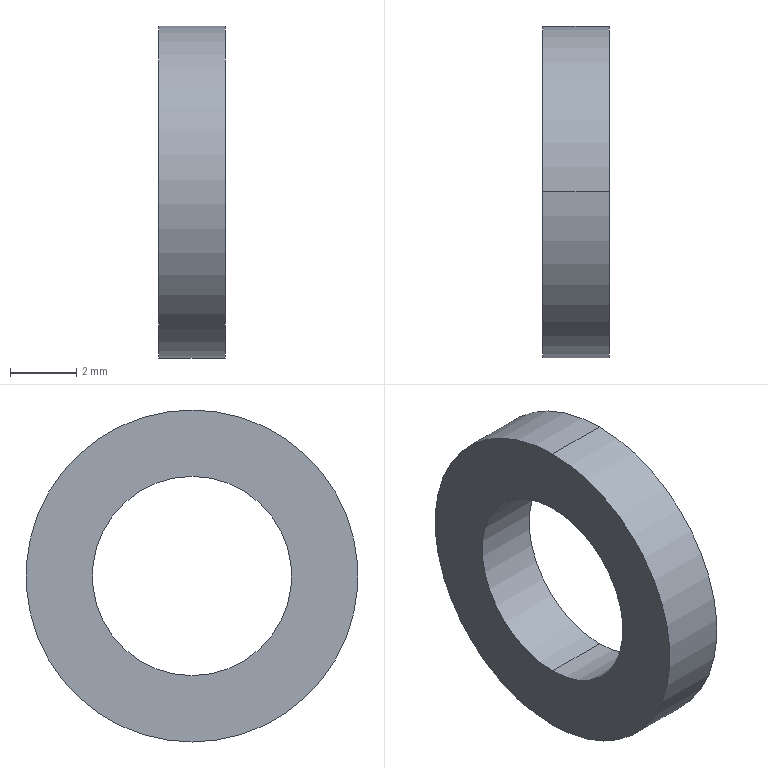Component | SolidWorks | A49-1 | 1 solid | 6 faces | box 2 x 10 x 10 mm | volume 101 mm3 | cylinder 4 | plane 2 | commonest cylinder face diameters 6 x2 10 x2 | material S45C
build123d program:
from build123d import *

# Parameters (mm, degrees)
SKETCH1_R           = 5
SKETCH1_R_2         = 3
BOSS_EXTRUDE1_DEPTH = 1


with BuildPart() as part:
    # Sketch1 → Boss-Extrude1 (new, symmetric)
    with BuildSketch(Plane(origin=(0, 0, 0), x_dir=(0, 0, -1), z_dir=(1, 0, 0))):
        Circle(SKETCH1_R)
        Circle(SKETCH1_R_2, mode=Mode.SUBTRACT)
    extrude(amount=BOSS_EXTRUDE1_DEPTH, both=True)


solid = part.part

# Placed as in the assembly
solid = solid.moved(Location((-16.351, 113.864, 5), (0, 0, 0)))
STEP:
#1=COLOUR_RGB('',0.7922,0.8196,0.9333);
#2=FILL_AREA_STYLE_COLOUR('',#1);
#3=FILL_AREA_STYLE('',(#2));
#4=SURFACE_STYLE_FILL_AREA(#3);
#5=SURFACE_SIDE_STYLE('',(#4));
#6=SURFACE_STYLE_USAGE(.BOTH.,#5);
#7=PRESENTATION_STYLE_ASSIGNMENT((#6));
#8=CARTESIAN_POINT('',(-0.6044,4.483,0.315));
#9=VERTEX_POINT('',#8);
#10=CARTESIAN_POINT('',(-0.6044,4.483,0.07874));
#11=VERTEX_POINT('',#10);
#12=CARTESIAN_POINT('',(-0.6044,4.483,0.1969));
#13=DIRECTION('',(1.,0.,0.));
#14=DIRECTION('',(0.,-0.,-1.));
#15=AXIS2_PLACEMENT_3D('',#12,#13,#14);
#16=CIRCLE('',#15,0.1181);
#17=EDGE_CURVE('',#9,#11,#16,.T.);
#18=ORIENTED_EDGE('',*,*,#17,.T.);
#19=CARTESIAN_POINT('',(-0.6831,4.483,0.07874));
#20=VERTEX_POINT('',#19);
#21=CARTESIAN_POINT('',(-0.6044,4.483,0.07874));
#22=DIRECTION('',(-1.,-0.,-0.));
#23=VECTOR('',#22,39.37);
#24=LINE('',#21,#23);
#25=EDGE_CURVE('',#11,#20,#24,.T.);
#26=ORIENTED_EDGE('',*,*,#25,.T.);
#27=CARTESIAN_POINT('',(-0.6831,4.483,0.315));
#28=VERTEX_POINT('',#27);
#29=CARTESIAN_POINT('',(-0.6831,4.483,0.1969));
#30=DIRECTION('',(1.,0.,0.));
#31=DIRECTION('',(0.,-0.,-1.));
#32=AXIS2_PLACEMENT_3D('',#29,#30,#31);
#33=CIRCLE('',#32,0.1181);
#34=EDGE_CURVE('',#28,#20,#33,.T.);
#35=ORIENTED_EDGE('',*,*,#34,.F.);
#36=CARTESIAN_POINT('',(-0.6044,4.483,0.315));
#37=DIRECTION('',(-1.,-0.,-0.));
#38=VECTOR('',#37,39.37);
#39=LINE('',#36,#38);
#40=EDGE_CURVE('',#9,#28,#39,.T.);
#41=ORIENTED_EDGE('',*,*,#40,.F.);
#42=EDGE_LOOP('',(#18,#26,#35,#41));
#43=FACE_OUTER_BOUND('',#42,.T.);
#44=CARTESIAN_POINT('',(-0.6044,4.483,0.1969));
#45=DIRECTION('',(-1.,-0.,-0.));
#46=DIRECTION('',(0.,0.,1.));
#47=AXIS2_PLACEMENT_3D('',#44,#45,#46);
#48=CYLINDRICAL_SURFACE('',#47,0.1181);
#49=ADVANCED_FACE('',(#43),#48,.F.);
#50=CARTESIAN_POINT('',(-0.6044,4.483,-0.));
#51=VERTEX_POINT('',#50);
#52=CARTESIAN_POINT('',(-0.6044,4.483,0.3937));
#53=VERTEX_POINT('',#52);
#54=CARTESIAN_POINT('',(-0.6044,4.483,0.1969));
#55=DIRECTION('',(1.,0.,0.));
#56=DIRECTION('',(0.,-0.,-1.));
#57=AXIS2_PLACEMENT_3D('',#54,#55,#56);
#58=CIRCLE('',#57,0.1969);
#59=EDGE_CURVE('',#51,#53,#58,.T.);
#60=ORIENTED_EDGE('',*,*,#59,.F.);
#61=CARTESIAN_POINT('',(-0.6831,4.483,-0.));
#62=VERTEX_POINT('',#61);
#63=CARTESIAN_POINT('',(-0.6044,4.483,-0.));
#64=DIRECTION('',(-1.,-0.,-0.));
#65=VECTOR('',#64,39.37);
#66=LINE('',#63,#65);
#67=EDGE_CURVE('',#51,#62,#66,.T.);
#68=ORIENTED_EDGE('',*,*,#67,.T.);
#69=CARTESIAN_POINT('',(-0.6831,4.483,0.3937));
#70=VERTEX_POINT('',#69);
#71=CARTESIAN_POINT('',(-0.6831,4.483,0.1969));
#72=DIRECTION('',(1.,0.,0.));
#73=DIRECTION('',(0.,-0.,-1.));
#74=AXIS2_PLACEMENT_3D('',#71,#72,#73);
#75=CIRCLE('',#74,0.1969);
#76=EDGE_CURVE('',#62,#70,#75,.T.);
#77=ORIENTED_EDGE('',*,*,#76,.T.);
#78=CARTESIAN_POINT('',(-0.6044,4.483,0.3937));
#79=DIRECTION('',(-1.,-0.,-0.));
#80=VECTOR('',#79,39.37);
#81=LINE('',#78,#80);
#82=EDGE_CURVE('',#53,#70,#81,.T.);
#83=ORIENTED_EDGE('',*,*,#82,.F.);
#84=EDGE_LOOP('',(#60,#68,#77,#83));
#85=FACE_OUTER_BOUND('',#84,.T.);
#86=CARTESIAN_POINT('',(-0.6044,4.483,0.1969));
#87=DIRECTION('',(-1.,-0.,-0.));
#88=DIRECTION('',(0.,0.,1.));
#89=AXIS2_PLACEMENT_3D('',#86,#87,#88);
#90=CYLINDRICAL_SURFACE('',#89,0.1969);
#91=ADVANCED_FACE('',(#85),#90,.T.);
#92=CARTESIAN_POINT('',(-0.6044,4.483,0.1969));
#93=DIRECTION('',(1.,0.,0.));
#94=DIRECTION('',(0.,-0.,-1.));
#95=AXIS2_PLACEMENT_3D('',#92,#93,#94);
#96=CIRCLE('',#95,0.1969);
#97=EDGE_CURVE('',#53,#51,#96,.T.);
#98=ORIENTED_EDGE('',*,*,#97,.T.);
#99=ORIENTED_EDGE('',*,*,#59,.T.);
#100=EDGE_LOOP('',(#98,#99));
#101=FACE_OUTER_BOUND('',#100,.T.);
#102=ORIENTED_EDGE('',*,*,#17,.F.);
#103=CARTESIAN_POINT('',(-0.6044,4.483,0.1969));
#104=DIRECTION('',(1.,0.,0.));
#105=DIRECTION('',(0.,-0.,-1.));
#106=AXIS2_PLACEMENT_3D('',#103,#104,#105);
#107=CIRCLE('',#106,0.1181);
#108=EDGE_CURVE('',#11,#9,#107,.T.);
#109=ORIENTED_EDGE('',*,*,#108,.F.);
#110=EDGE_LOOP('',(#102,#109));
#111=FACE_BOUND('',#110,.T.);
#112=CARTESIAN_POINT('',(-0.6044,4.483,0.1969));
#113=DIRECTION('',(1.,0.,0.));
#114=DIRECTION('',(0.,-0.,-1.));
#115=AXIS2_PLACEMENT_3D('',#112,#113,#114);
#116=PLANE('',#115);
#117=ADVANCED_FACE('',(#101,#111),#116,.T.);
#118=CARTESIAN_POINT('',(-0.6831,4.483,0.1969));
#119=DIRECTION('',(1.,0.,0.));
#120=DIRECTION('',(0.,-0.,-1.));
#121=AXIS2_PLACEMENT_3D('',#118,#119,#120);
#122=CIRCLE('',#121,0.1969);
#123=EDGE_CURVE('',#70,#62,#122,.T.);
#124=ORIENTED_EDGE('',*,*,#123,.F.);
#125=ORIENTED_EDGE('',*,*,#76,.F.);
#126=EDGE_LOOP('',(#124,#125));
#127=FACE_OUTER_BOUND('',#126,.T.);
#128=ORIENTED_EDGE('',*,*,#34,.T.);
#129=CARTESIAN_POINT('',(-0.6831,4.483,0.1969));
#130=DIRECTION('',(1.,0.,0.));
#131=DIRECTION('',(0.,-0.,-1.));
#132=AXIS2_PLACEMENT_3D('',#129,#130,#131);
#133=CIRCLE('',#132,0.1181);
#134=EDGE_CURVE('',#20,#28,#133,.T.);
#135=ORIENTED_EDGE('',*,*,#134,.T.);
#136=EDGE_LOOP('',(#128,#135));
#137=FACE_BOUND('',#136,.T.);
#138=CARTESIAN_POINT('',(-0.6831,4.483,0.1969));
#139=DIRECTION('',(1.,0.,0.));
#140=DIRECTION('',(0.,-0.,-1.));
#141=AXIS2_PLACEMENT_3D('',#138,#139,#140);
#142=PLANE('',#141);
#143=ADVANCED_FACE('',(#127,#137),#142,.F.);
#144=ORIENTED_EDGE('',*,*,#67,.F.);
#145=ORIENTED_EDGE('',*,*,#97,.F.);
#146=ORIENTED_EDGE('',*,*,#82,.T.);
#147=ORIENTED_EDGE('',*,*,#123,.T.);
#148=EDGE_LOOP('',(#144,#145,#146,#147));
#149=FACE_OUTER_BOUND('',#148,.T.);
#150=CARTESIAN_POINT('',(-0.6044,4.483,0.1969));
#151=DIRECTION('',(-1.,-0.,-0.));
#152=DIRECTION('',(0.,0.,1.));
#153=AXIS2_PLACEMENT_3D('',#150,#151,#152);
#154=CYLINDRICAL_SURFACE('',#153,0.1969);
#155=ADVANCED_FACE('',(#149),#154,.T.);
#156=ORIENTED_EDGE('',*,*,#25,.F.);
#157=ORIENTED_EDGE('',*,*,#108,.T.);
#158=ORIENTED_EDGE('',*,*,#40,.T.);
#159=ORIENTED_EDGE('',*,*,#134,.F.);
#160=EDGE_LOOP('',(#156,#157,#158,#159));
#161=FACE_OUTER_BOUND('',#160,.T.);
#162=CARTESIAN_POINT('',(-0.6044,4.483,0.1969));
#163=DIRECTION('',(-1.,-0.,-0.));
#164=DIRECTION('',(0.,0.,1.));
#165=AXIS2_PLACEMENT_3D('',#162,#163,#164);
#166=CYLINDRICAL_SURFACE('',#165,0.1181);
#167=ADVANCED_FACE('',(#161),#166,.F.);
#168=CLOSED_SHELL('',(#49,#91,#117,#143,#155,#167));
#169=MANIFOLD_SOLID_BREP('',#168);
#170=STYLED_ITEM('',(#7),#169);
#171=(LENGTH_UNIT()NAMED_UNIT(*)SI_UNIT($,.METRE.));
#172=LENGTH_MEASURE_WITH_UNIT(LENGTH_MEASURE(0.0254),#171);
#173=DIMENSIONAL_EXPONENTS(1.,0.,0.,0.,0.,0.,0.);
#174=(CONVERSION_BASED_UNIT('',#172)LENGTH_UNIT()NAMED_UNIT(#173));
#175=UNCERTAINTY_MEASURE_WITH_UNIT(LENGTH_MEASURE(0.00001),#174,'','');
#176=(NAMED_UNIT(*)PLANE_ANGLE_UNIT()SI_UNIT($,.RADIAN.));
#177=(NAMED_UNIT(*)SI_UNIT($,.STERADIAN.)SOLID_ANGLE_UNIT());
#178=(GEOMETRIC_REPRESENTATION_CONTEXT(3)GLOBAL_UNCERTAINTY_ASSIGNED_CONTEXT((#175))GLOBAL_UNIT_ASSIGNED_CONTEXT((#174,#176,#177))REPRESENTATION_CONTEXT('',''));
#179=MECHANICAL_DESIGN_GEOMETRIC_PRESENTATION_REPRESENTATION('',(#170),#178);
#180=CARTESIAN_POINT('',(0.,0.,0.));
#181=DIRECTION('',(0.,0.,1.));
#182=DIRECTION('',(1.,0.,0.));
#183=AXIS2_PLACEMENT_3D('',#180,#181,#182);
#184=(LENGTH_UNIT()NAMED_UNIT(*)SI_UNIT($,.METRE.));
#185=LENGTH_MEASURE_WITH_UNIT(LENGTH_MEASURE(0.0254),#184);
#186=DIMENSIONAL_EXPONENTS(1.,0.,0.,0.,0.,0.,0.);
#187=(CONVERSION_BASED_UNIT('',#185)LENGTH_UNIT()NAMED_UNIT(#186));
#188=UNCERTAINTY_MEASURE_WITH_UNIT(LENGTH_MEASURE(0.00001),#187,'','');
#189=(NAMED_UNIT(*)PLANE_ANGLE_UNIT()SI_UNIT($,.RADIAN.));
#190=(NAMED_UNIT(*)SI_UNIT($,.STERADIAN.)SOLID_ANGLE_UNIT());
#191=(GEOMETRIC_REPRESENTATION_CONTEXT(3)GLOBAL_UNCERTAINTY_ASSIGNED_CONTEXT((#188))GLOBAL_UNIT_ASSIGNED_CONTEXT((#187,#189,#190))REPRESENTATION_CONTEXT('',''));
#192=ADVANCED_BREP_SHAPE_REPRESENTATION('',(#169,#183),#191);
#193=PRESENTATION_LAYER_ASSIGNMENT('','',(#170));